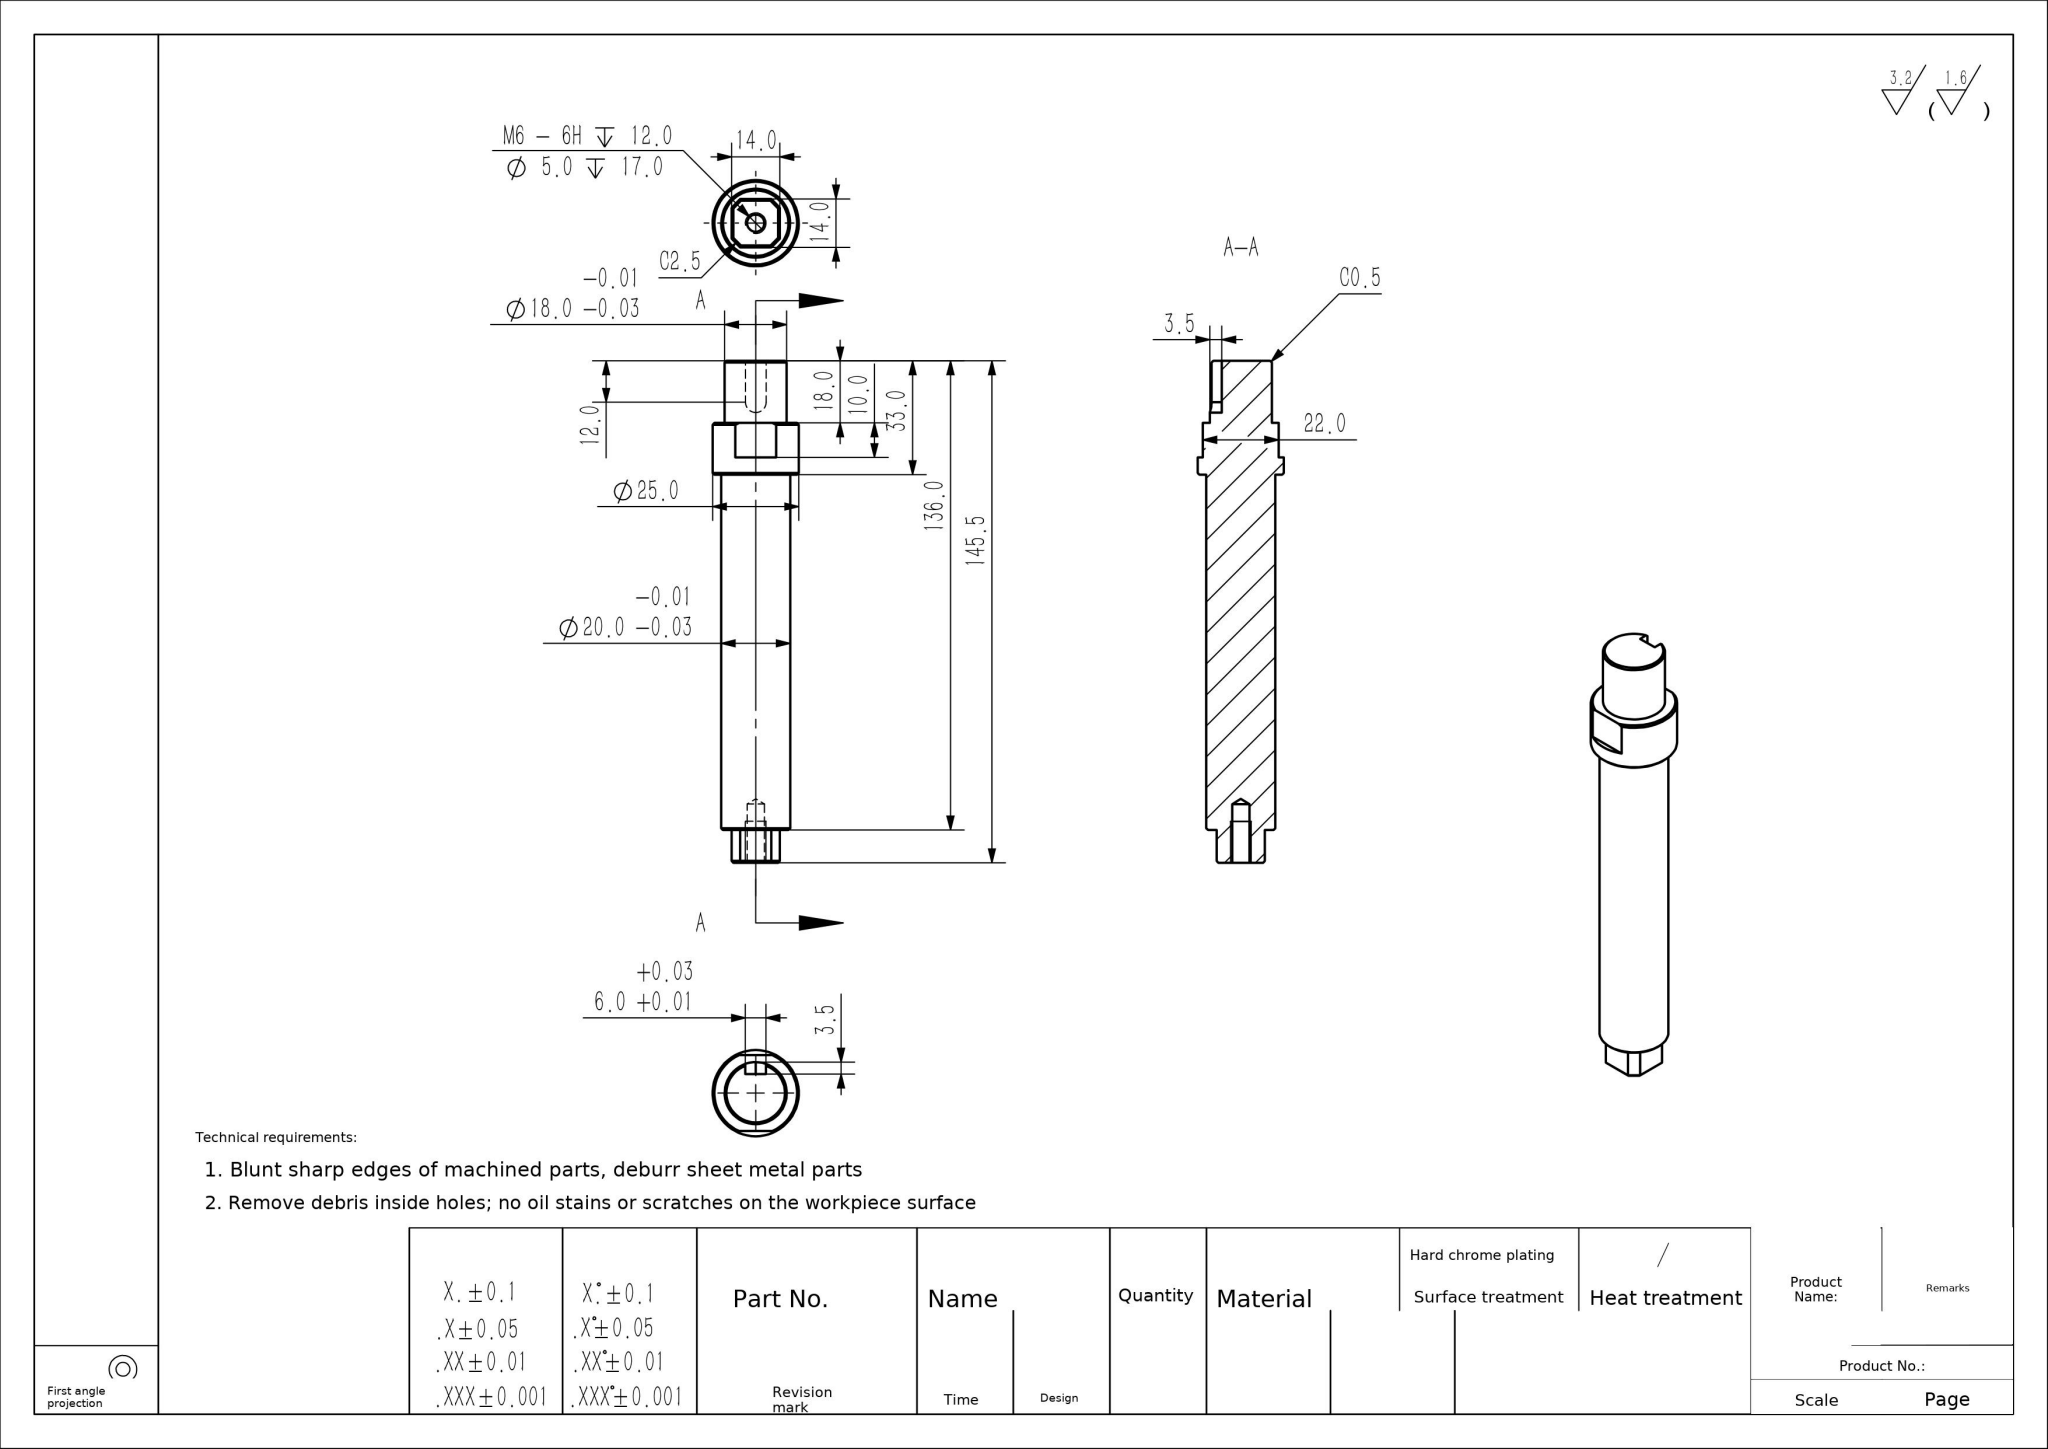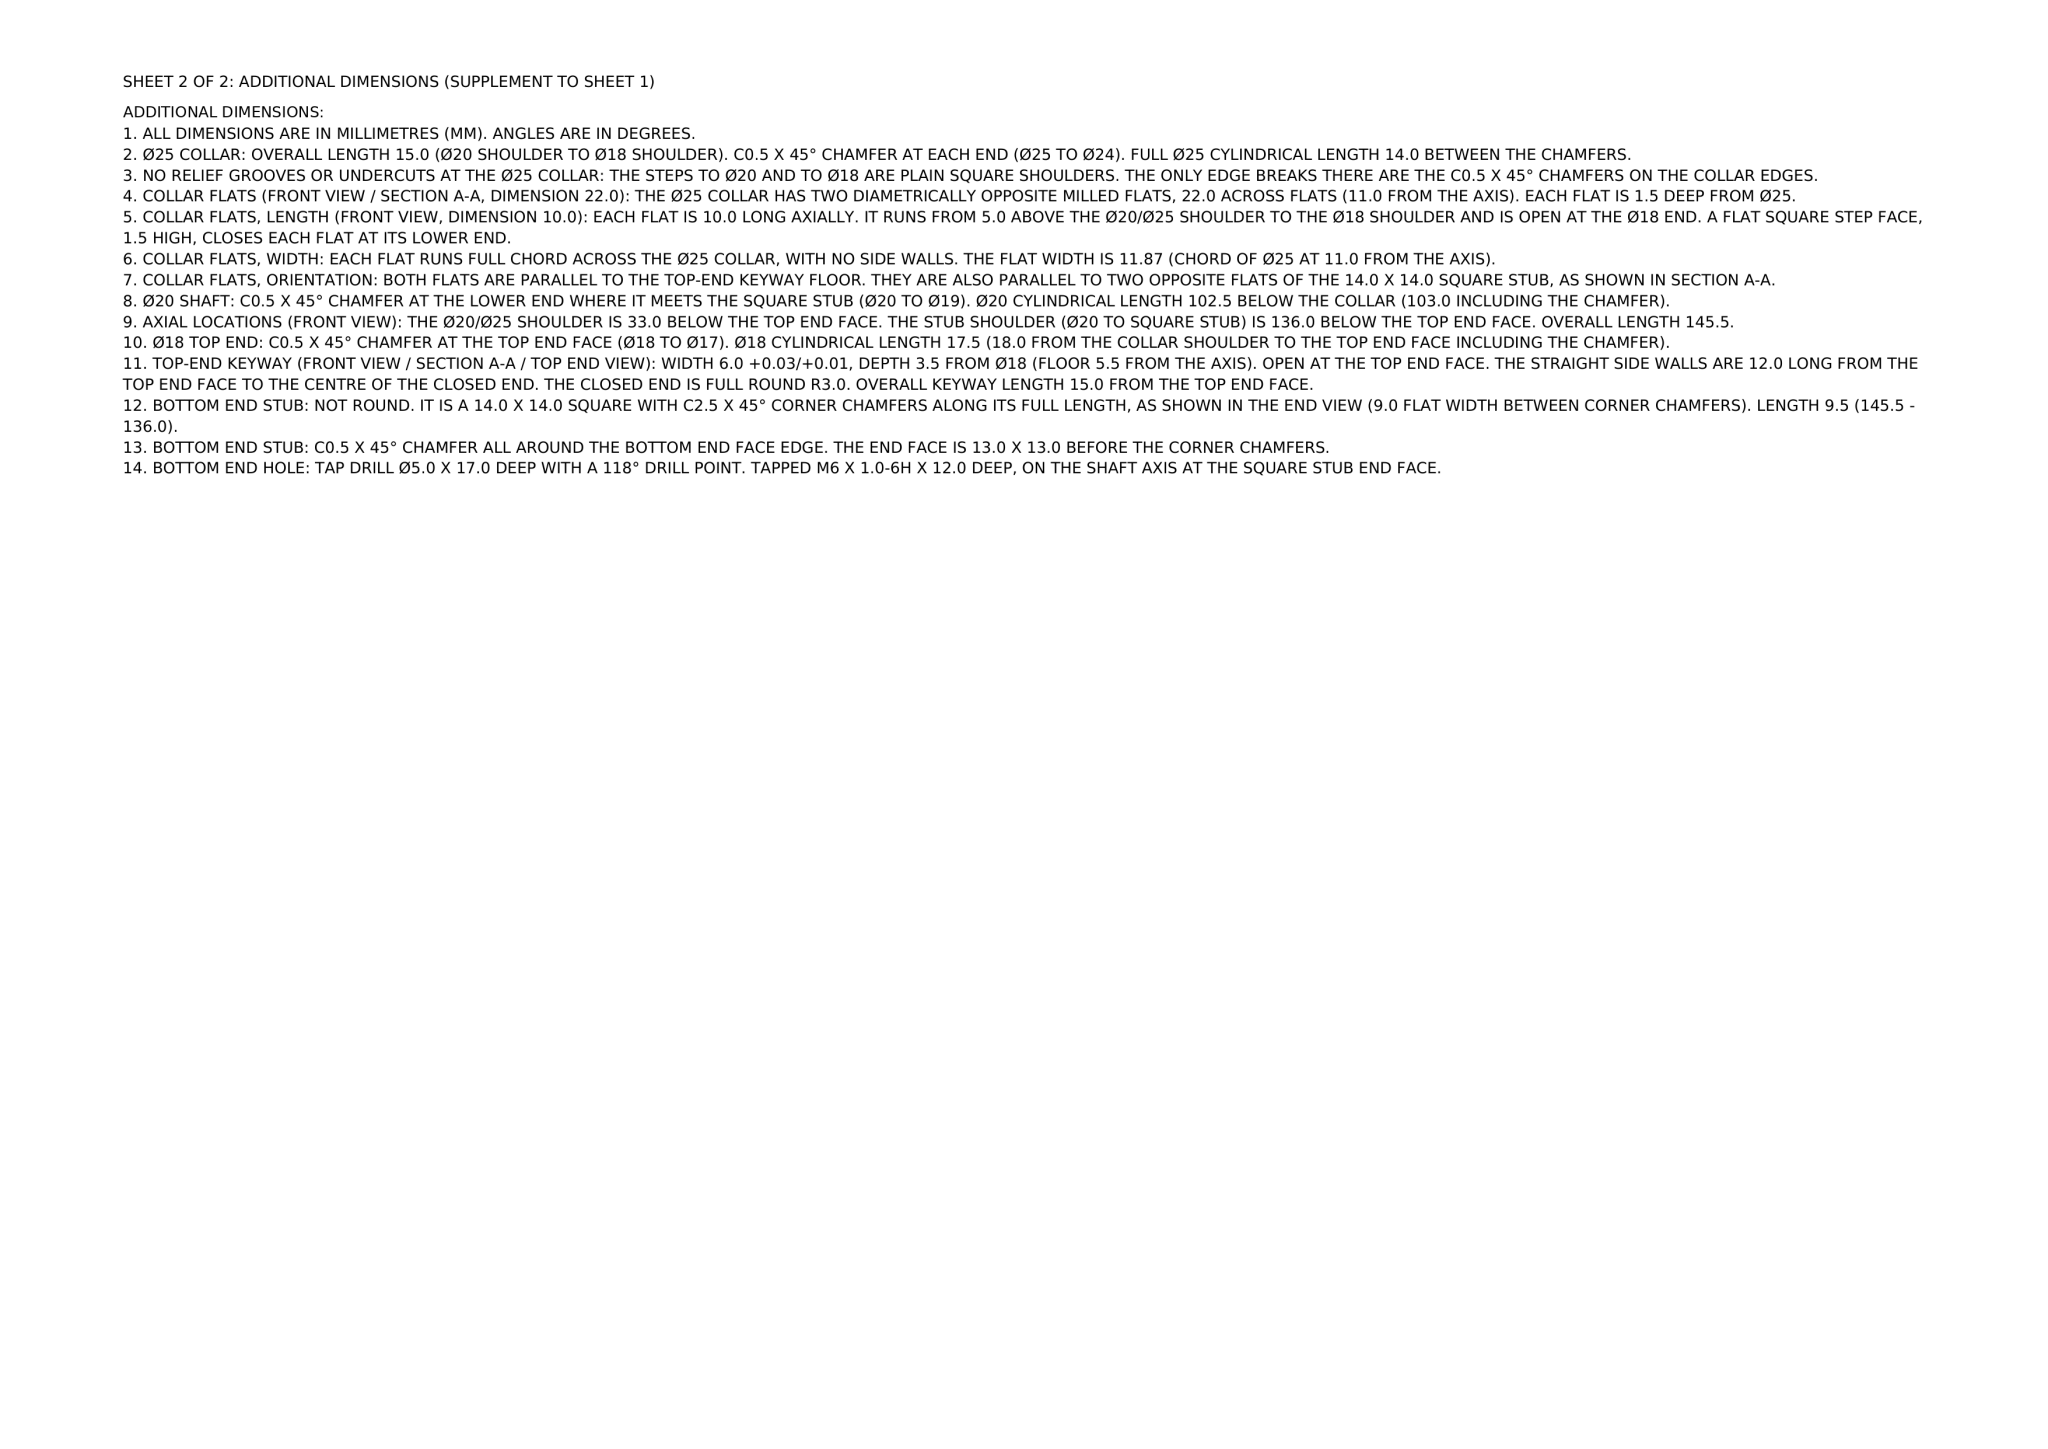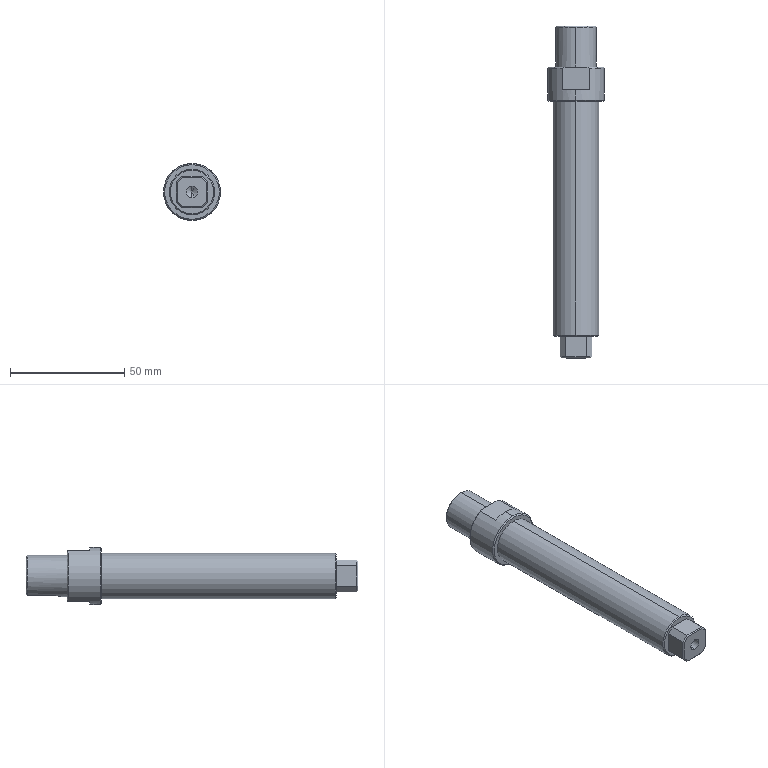Part | NX | mm | 1 solid | 47 faces | box 25 x 145.5 x 25 mm | volume 45137 mm3 | plane 28 | cylinder 10 | cone 9 | commonest cylinder face diameters 5 x2 20 x2 18 x2 25 x2 6 x2